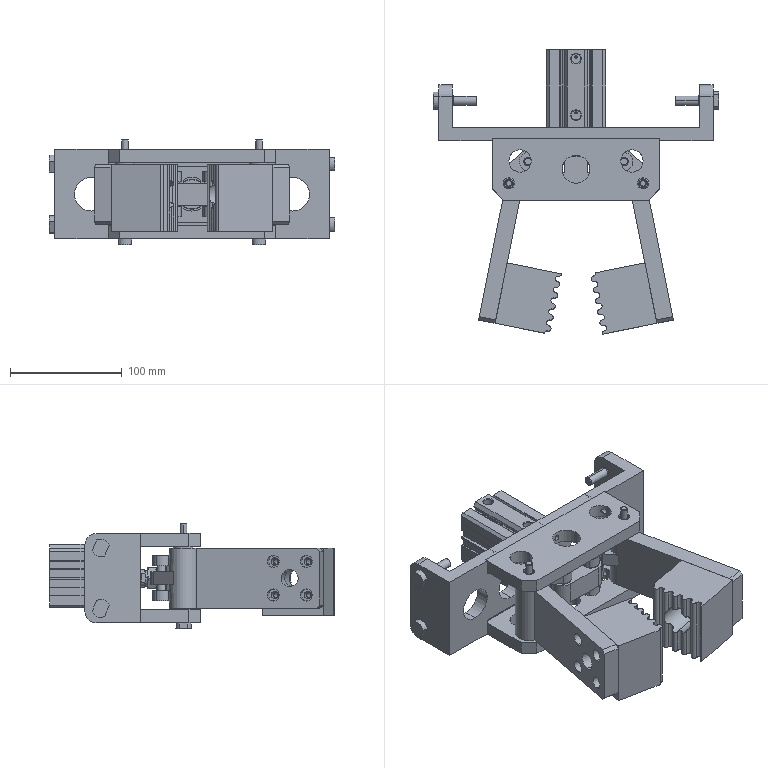Assembly | SolidWorks | mm | 29 component files | 29 solids | 997 faces | box 255 x 254.37 x 94 mm | volume 1114562 mm3 | cylinder 479 | plane 296 | cone 190 | torus 32 | commonest cylinder face diameters 5 x79 11 x40 10 x40 6.6 x36 8 x36 0.4 x35 16 x24 12 x24
Bill of materials:
ZTDJ-L-400-04-24-MaterialPortBagClamp-T-shapedConnectingRod | 1 | 1023 Carbon Steel Sheet (SS) | Prismatic block: an obround (stadium-shaped) body with two vertical through holes, one near each rounded end, plus a rectangular lug sticking out from one long side between the holes. The lug and the obround body look the same height.
C-SFF10120 | 4 | Tin Bronze | Flanged cylindrical sleeve: a thin circular flange on top of a straight cylindrical body, with one through bore along the axis.
MPBZ8_20 | 2 |  | Plain hollow cylindrical sleeve/tube with a straight through-bore and chamfered end edges; length roughly 1.6 times the outer diameter, and the bore is roughly two-thirds of the outer diameter (proportions estimated from the renders).
ZTDJ-01-20-AxisMountingPlate | 2 | 1023 Carbon Steel Sheet (SS) | Thin flat rectangular plate with two corners chamfered along one long edge. It has three large through holes in a row (the centre one is biggest) and two small through holes near the chamfered corners.
ZTDJ-L-400-04-16-MaterialPortBagClamp-Axis4 | 4 | 1023 Carbon Steel Sheet (SS) | Stepped cylindrical pin or shaft: a long smaller-diameter shank, a shorter larger-diameter section, and an end head that is wider still and has two parallel flats.
ZTDJ-L-400-04-19-MaterialPortBagClamp-ConnectingRodSeat2 | 1 | 1023 Carbon Steel Sheet (SS) | U-shaped channel bracket: a long rectangular web with a short perpendicular flange at each end. The web has five large through holes in a row and several small holes. Each flange has two holes and rounded outer corners.
ZTDJ-L-400-04-21-MaterialPortBagClamp-Axis5 | 2 | 1023 Carbon Steel Sheet (SS) | Slender stepped pin: a long main cylindrical body, a short smaller-diameter spigot at one end, and a wider collar or head at the other end with flats on its outline.
ZTDJ-L-400-04-22-MaterialPortBagClamp-BagClampingArm | 2 | 1023 Carbon Steel Sheet (SS) | Arm or lever-like bar: a long rectangular-section body with a round boss at one end carrying a through hole. A pattern of holes near the other end includes a larger central hole and four smaller holes, which appear counterbored.
ZTDJ-L-400-04-23-MaterialPortBagClamp-H-shapedConnectingRod | 2 | 1023 Carbon Steel Sheet (SS) | H-shaped part: two parallel obround plates, each with two through holes near the rounded ends, joined by a central rectangular web.
ZTDJ-L-400-04-25-MaterialPortBagClamp-Axis6 | 4 | Alloy Steel | Plain cylindrical pin with chamfered ends and two small radial holes, one near each end, on the same side.
ZTDJ-L-400-04-26-MaterialPortBagClamp-BagClampingAluminumBlock | 2 | 6061-T6 (SS) | Rectangular block with a row of semicircular scallops along one edge (they run as grooves along its full length). One face has a large round through bore with four small holes in a square pattern around it.
Mates:
1. coincident | ZTDJ-L-400-04-19-MaterialPortBagClamp-ConnectingRodSeat2-1 face at (-28.439, -44.186, 290) dir (0, -1, 0) | ZTDJ-01-20-AxisMountingPlate-1 face at (-103.439, -44.186, 330) dir (0, 1, 0)
2. coincident | ZTDJ-L-400-04-19-MaterialPortBagClamp-ConnectingRodSeat2-1 plane at (-28.439, -46.186, 290) dir (1, 0, 0) | ZTDJ-01-20-AxisMountingPlate-1 plane at (-28.439, -71.686, 324) dir (1, 0, 0)
3. coincident | ZTDJ-L-400-04-19-MaterialPortBagClamp-ConnectingRodSeat2-1 face at (-28.439, -44.186, 290) dir (0, -1, 0) | ZTDJ-01-20-AxisMountingPlate-2 face at (-103.439, -44.186, 262) dir (0, 1, 0)
4. coincident | ZTDJ-L-400-04-19-MaterialPortBagClamp-ConnectingRodSeat2-1 plane at (-28.439, -46.186, 290) dir (1, 0, 0) | ZTDJ-01-20-AxisMountingPlate-2 plane at (-28.439, -71.686, 256) dir (1, 0, 0)
5. concentric | ZTDJ-01-20-AxisMountingPlate-1 face at (31.561, -84.186, 318) dir (0, 0, 1) r 5 | ZTDJ-L-400-04-22-MaterialPortBagClamp-BagClampingArm-1 face at (31.561, -84.186, 263) dir (0, 0, 1) r 5.5
6. concentric | ZTDJ-01-20-AxisMountingPlate-2 face at (-88.439, -84.186, 250) dir (0, 0, 1) r 5 | ZTDJ-L-400-04-22-MaterialPortBagClamp-BagClampingArm-2 face at (-88.439, -84.186, 317) dir (0, 0, -1) r 5.5
7. concentric | ZTDJ-L-400-04-23-MaterialPortBagClamp-H-shapedConnectingRod-2 face at (-71.256, -64.673, 310) dir (0, 0, -1) r 4 | ZTDJ-L-400-04-22-MaterialPortBagClamp-BagClampingArm-2 face at (-71.256, -64.673, 296) dir (0, 0, -1) r 5
8. concentric | ZTDJ-L-400-04-19-MaterialPortBagClamp-ConnectingRodSeat2-1 face at (-28.439, 3.814, 290) dir (0, -1, 0) r 15 | ACQ40x30SB(0)+()-1/ACQS-40x30-B_30r-1 face at (-28.439, 18.755, 290) dir (0, -1, 0) r 8
9. coincident | ZTDJ-L-400-04-19-MaterialPortBagClamp-ConnectingRodSeat2-1 face at (-28.439, -34.186, 290) dir (0, 1, 0) | ACQ40x30SB(0)+()-1/ACQS-40x3030_b-1 face at (-20.039, -34.186, 264.2) dir (0, -1, 0)
10. coincident | ZTDJ-L-400-04-19-MaterialPortBagClamp-ConnectingRodSeat2-1 face at (-150.939, -34.186, 250) dir (0, 0, -1) | ZTDJ-01-20-AxisMountingPlate-2 face at (-28.439, -71.686, 250) dir (0, 0, -1)
11. coincident | ZTDJ-L-400-04-19-MaterialPortBagClamp-ConnectingRodSeat2-1 face at (34.061, -34.186, 330) dir (0, 0, 1) | ZTDJ-01-20-AxisMountingPlate-1 face at (-28.439, -71.686, 330) dir (0, 0, 1)
12. concentric | ZTDJ-L-400-04-23-MaterialPortBagClamp-H-shapedConnectingRod-2 face at (-45.939, -84.245, 310) dir (0, 0, -1) r 4 | ACQ40x30SB(0)+()-1/ZTDJ-L-400-04-24-MaterialPortBagClamp-T-shapedConnectingRod-2 face at (-45.939, -84.245, 300) dir (0, 0, -1) r 6
13. concentric | ZTDJ-L-400-04-23-MaterialPortBagClamp-H-shapedConnectingRod-1 face at (-10.939, -84.245, 310) dir (0, 0, -1) r 4 | ACQ40x30SB(0)+()-1/ZTDJ-L-400-04-24-MaterialPortBagClamp-T-shapedConnectingRod-2 face at (-10.939, -84.245, 300) dir (0, 0, -1) r 6
14. concentric | ZTDJ-L-400-04-22-MaterialPortBagClamp-BagClampingArm-1 face at (14.378, -64.673, 284) dir (0, 0, 1) r 5 | ZTDJ-L-400-04-23-MaterialPortBagClamp-H-shapedConnectingRod-1 face at (14.378, -64.673, 310) dir (0, 0, -1) r 4
15. distance | ZTDJ-L-400-04-23-MaterialPortBagClamp-H-shapedConnectingRod-2 face at (-82.478, -66.11, 279) dir (0, 0, 1) | ACQ40x30SB(0)+()-1/ZTDJ-L-400-04-24-MaterialPortBagClamp-T-shapedConnectingRod-2 face at (-45.939, -84.245, 280) dir (0, 0, -1)
16. coincident | ZTDJ-L-400-04-23-MaterialPortBagClamp-H-shapedConnectingRod-1 face at (-10.939, -84.245, 270) dir (0, 0, -1) | ZTDJ-L-400-04-23-MaterialPortBagClamp-H-shapedConnectingRod-2 face at (-71.256, -64.673, 270) dir (0, 0, -1)
17. concentric | ZTDJ-L-400-04-19-MaterialPortBagClamp-ConnectingRodSeat2-1 face at (-150.939, -10.186, 263) dir (1, 0, 0) r 5 | ZTDJ-L-400-04-16-MaterialPortBagClamp-Axis4-4 face at (-150.939, -10.186, 263) dir (1, 0, 0) r 5
18. coincident | ZTDJ-L-400-04-19-MaterialPortBagClamp-ConnectingRodSeat2-1 face at (-150.939, -34.186, 330) dir (-1, 0, 0) | ZTDJ-L-400-04-16-MaterialPortBagClamp-Axis4-4 face at (-150.939, -10.186, 263) dir (1, 0, 0)
19. concentric | ZTDJ-L-400-04-19-MaterialPortBagClamp-ConnectingRodSeat2-1 face at (-150.939, -10.186, 317) dir (1, 0, 0) r 5 | ZTDJ-L-400-04-16-MaterialPortBagClamp-Axis4-3 face at (-150.939, -10.186, 317) dir (1, 0, 0) r 5
20. coincident | ZTDJ-L-400-04-16-MaterialPortBagClamp-Axis4-3 face at (-155.939, -10.186, 317) dir (-1, 0, 0) | ZTDJ-L-400-04-16-MaterialPortBagClamp-Axis4-4 face at (-155.939, -10.186, 263) dir (-1, 0, 0)
21. concentric | ZTDJ-L-400-04-19-MaterialPortBagClamp-ConnectingRodSeat2-1 face at (-150.939, -10.186, 263) dir (1, 0, 0) r 5 | ZTDJ-L-400-04-16-MaterialPortBagClamp-Axis4-2 face at (94.061, -10.186, 263) dir (-1, 0, 0) r 5
22. concentric | ZTDJ-L-400-04-19-MaterialPortBagClamp-ConnectingRodSeat2-1 face at (-150.939, -10.186, 317) dir (1, 0, 0) r 5 | ZTDJ-L-400-04-16-MaterialPortBagClamp-Axis4-1 face at (94.061, -10.186, 317) dir (-1, 0, 0) r 5
23. coincident | ZTDJ-L-400-04-19-MaterialPortBagClamp-ConnectingRodSeat2-1 face at (94.061, -34.186, 330) dir (1, 0, 0) | ZTDJ-L-400-04-16-MaterialPortBagClamp-Axis4-2 face at (94.061, -10.186, 263) dir (-1, 0, 0)
24. coincident | ZTDJ-L-400-04-19-MaterialPortBagClamp-ConnectingRodSeat2-1 face at (94.061, -34.186, 330) dir (1, 0, 0) | ZTDJ-L-400-04-16-MaterialPortBagClamp-Axis4-1 face at (94.061, -10.186, 317) dir (-1, 0, 0)
25. concentric | ACQ40x30SB(0)+()-1/ZTDJ-L-400-04-24-MaterialPortBagClamp-T-shapedConnectingRod-2 face at (-10.939, -84.245, 300) dir (0, 0, -1) r 6 | MPBZ8_20-1 face at (-10.939, -84.245, 280) dir (0, 0, 1) r 6
26. coincident | ACQ40x30SB(0)+()-1/ZTDJ-L-400-04-24-MaterialPortBagClamp-T-shapedConnectingRod-2 face at (-45.939, -84.245, 300) dir (0, 0, 1) | MPBZ8_20-1 face at (-15.171, -88.063, 300) dir (0, 0, 1)
27. concentric | ACQ40x30SB(0)+()-1/ZTDJ-L-400-04-24-MaterialPortBagClamp-T-shapedConnectingRod-2 face at (-45.939, -84.245, 300) dir (0, 0, -1) r 6 | MPBZ8_20-2 face at (-45.939, -84.245, 280) dir (0, 0, 1) r 6
28. coincident | ACQ40x30SB(0)+()-1/ZTDJ-L-400-04-24-MaterialPortBagClamp-T-shapedConnectingRod-2 face at (-45.939, -84.245, 300) dir (0, 0, 1) | MPBZ8_20-2 face at (-46.858, -78.62, 300) dir (0, 0, 1)
29. concentric | ZTDJ-L-400-04-23-MaterialPortBagClamp-H-shapedConnectingRod-1 face at (14.378, -64.673, 310) dir (0, 0, -1) r 4 | ZTDJ-L-400-04-25-MaterialPortBagClamp-Axis6-1 face at (14.378, -64.673, 310) dir (0, 0, -1) r 4
30. concentric | ZTDJ-L-400-04-23-MaterialPortBagClamp-H-shapedConnectingRod-1 face at (-10.939, -84.245, 310) dir (0, 0, -1) r 4 | ZTDJ-L-400-04-25-MaterialPortBagClamp-Axis6-2 face at (-10.939, -84.245, 310) dir (0, 0, -1) r 4
31. concentric | ZTDJ-L-400-04-23-MaterialPortBagClamp-H-shapedConnectingRod-2 face at (-45.939, -84.245, 310) dir (0, 0, -1) r 4 | ZTDJ-L-400-04-25-MaterialPortBagClamp-Axis6-3 face at (-45.939, -84.245, 310) dir (0, 0, -1) r 4
32. concentric | ZTDJ-L-400-04-23-MaterialPortBagClamp-H-shapedConnectingRod-2 face at (-71.256, -64.673, 310) dir (0, 0, -1) r 4 | ZTDJ-L-400-04-25-MaterialPortBagClamp-Axis6-4 face at (-71.256, -64.673, 310) dir (0, 0, -1) r 4
33. concentric | ZTDJ-01-20-AxisMountingPlate-2 face at (31.561, -84.186, 250) dir (0, 0, 1) r 5 | ZTDJ-L-400-04-21-MaterialPortBagClamp-Axis5-1 face at (31.561, -84.186, 329) dir (0, 0, -1) r 5
34. coincident | ZTDJ-01-20-AxisMountingPlate-2 face at (-28.439, -71.686, 250) dir (0, 0, -1) | ZTDJ-L-400-04-21-MaterialPortBagClamp-Axis5-1 face at (31.561, -84.186, 250) dir (0, 0, 1)
35. concentric | ZTDJ-01-20-AxisMountingPlate-1 face at (-88.439, -84.186, 318) dir (0, 0, 1) r 5 | ZTDJ-L-400-04-21-MaterialPortBagClamp-Axis5-2 face at (-88.439, -84.186, 329) dir (0, 0, -1) r 5
36. coincident | ZTDJ-01-20-AxisMountingPlate-2 face at (-28.439, -71.686, 250) dir (0, 0, -1) | ZTDJ-L-400-04-21-MaterialPortBagClamp-Axis5-2 face at (-88.439, -84.186, 250) dir (0, 0, 1)
37. coincident | ZTDJ-L-400-04-22-MaterialPortBagClamp-BagClampingArm-1 face at (22.263, -101.355, 137.103) dir (-0.9804, -0.1971, 0) | ZTDJ-L-400-04-26-MaterialPortBagClamp-BagClampingAluminumBlock-1 face at (33.103, -155.277, 257) dir (0.9804, 0.1971, 0)
38. coincident | ZTDJ-L-400-04-22-MaterialPortBagClamp-BagClampingArm-2 face at (-79.141, -101.355, 442.897) dir (0.9804, -0.1971, 0) | ZTDJ-L-400-04-26-MaterialPortBagClamp-BagClampingAluminumBlock-2 face at (-100.821, -209.198, 257) dir (-0.9804, 0.1971, 0)
39. coincident | ZTDJ-L-400-04-22-MaterialPortBagClamp-BagClampingArm-2 face at (-88.439, -84.186, 317) dir (0, 0, 1) | ZTDJ-L-400-04-26-MaterialPortBagClamp-BagClampingAluminumBlock-2 face at (-72.117, -186.918, 317) dir (0, 0, 1)
40. distance | ZTDJ-L-400-04-22-MaterialPortBagClamp-BagClampingArm-2 face at (-100.821, -209.198, 442.897) dir (-0.1971, -0.9804, 0) | ZTDJ-L-400-04-26-MaterialPortBagClamp-BagClampingAluminumBlock-2 face at (-54.253, -218.56, 257) dir (-0.1971, -0.9804, 0)
41. concentric | ZTDJ-L-400-04-22-MaterialPortBagClamp-BagClampingArm-1 face at (31.561, -84.186, 302) dir (0, 0, 1) r 6 | C-SFF10120-1 face at (31.561, -84.186, 318) dir (0, 0, 1) r 6
42. coincident | ZTDJ-L-400-04-22-MaterialPortBagClamp-BagClampingArm-1 face at (31.561, -84.186, 317) dir (0, 0, 1) | C-SFF10120-1 face at (31.561, -75.186, 317) dir (0, 0, -1)
43. concentric | ZTDJ-L-400-04-22-MaterialPortBagClamp-BagClampingArm-1 face at (31.561, -84.186, 278) dir (0, 0, -1) r 6 | C-SFF10120-2 face at (31.561, -84.186, 262) dir (0, 0, -1) r 6
44. coincident | ZTDJ-L-400-04-22-MaterialPortBagClamp-BagClampingArm-1 face at (31.561, -84.186, 263) dir (0, 0, -1) | C-SFF10120-2 face at (28.114, -75.872, 263) dir (0, 0, 1)
45. coincident | ZTDJ-L-400-04-22-MaterialPortBagClamp-BagClampingArm-2 face at (-88.439, -84.186, 263) dir (0, 0, -1) | C-SFF10120-3 face at (-91.886, -75.872, 263) dir (0, 0, 1)
46. concentric | ZTDJ-L-400-04-22-MaterialPortBagClamp-BagClampingArm-2 face at (-88.439, -84.186, 278) dir (0, 0, -1) r 6 | C-SFF10120-3 face at (-88.439, -84.186, 262) dir (0, 0, -1) r 6
47. coincident | ZTDJ-L-400-04-22-MaterialPortBagClamp-BagClampingArm-2 face at (-88.439, -84.186, 317) dir (0, 0, 1) | C-SFF10120-4 face at (-88.439, -75.186, 317) dir (0, 0, -1)
48. concentric | ZTDJ-L-400-04-22-MaterialPortBagClamp-BagClampingArm-2 face at (-88.439, -84.186, 302) dir (0, 0, 1) r 6 | C-SFF10120-4 face at (-88.439, -84.186, 318) dir (0, 0, 1) r 6
49. coincident | ZTDJ-01-20-AxisMountingPlate-2 face at (-28.439, -71.686, 262) dir (0, 0, 1) | C-SFF10120-3 face at (-90.354, -79.567, 262) dir (0, 0, -1)
50. coincident | ZTDJ-01-20-AxisMountingPlate-1 face at (-28.439, -71.686, 318) dir (0, 0, -1) | C-SFF10120-1 face at (31.561, -79.186, 318) dir (0, 0, 1)
51. coincident | ZTDJ-L-400-04-22-MaterialPortBagClamp-BagClampingArm-1 face at (43.944, -209.198, 137.103) dir (0.1971, -0.9804, 0) | ZTDJ-L-400-04-26-MaterialPortBagClamp-BagClampingAluminumBlock-1 face at (-2.625, -218.56, 257) dir (0.1971, -0.9804, 0)
52. coincident | ZTDJ-L-400-04-22-MaterialPortBagClamp-BagClampingArm-1 face at (31.561, -84.186, 317) dir (0, 0, 1) | ZTDJ-L-400-04-26-MaterialPortBagClamp-BagClampingAluminumBlock-1 face at (15.239, -186.918, 317) dir (0, 0, 1)
53. coincident | ZTDJ-L-400-04-23-MaterialPortBagClamp-H-shapedConnectingRod-1 face at (-10.939, -84.245, 270) dir (0, 0, -1) | ZTDJ-L-400-04-25-MaterialPortBagClamp-Axis6-1 face at (14.378, -64.673, 270) dir (0, 0, -1)
54. coincident | ZTDJ-L-400-04-23-MaterialPortBagClamp-H-shapedConnectingRod-2 face at (-71.256, -64.673, 270) dir (0, 0, -1) | ZTDJ-L-400-04-25-MaterialPortBagClamp-Axis6-4 face at (-71.256, -64.673, 270) dir (0, 0, -1)
55. coincident | ZTDJ-L-400-04-23-MaterialPortBagClamp-H-shapedConnectingRod-2 face at (-71.256, -64.673, 270) dir (0, 0, -1) | ZTDJ-L-400-04-25-MaterialPortBagClamp-Axis6-3 face at (-45.939, -84.245, 270) dir (0, 0, -1)
56. coincident | ZTDJ-L-400-04-23-MaterialPortBagClamp-H-shapedConnectingRod-1 face at (-10.939, -84.245, 270) dir (0, 0, -1) | ZTDJ-L-400-04-25-MaterialPortBagClamp-Axis6-2 face at (-10.939, -84.245, 270) dir (0, 0, -1)
57. distance | ACQS-40x30-B_30r-1 face at (-58.5, 0, 0) dir (-1, 0, 0) | ACQS-40x3030_b-1 face at (0, -8.4, -25.8) dir (-1, 0, 0)
58. concentric | ACQS-40x3030_b-1 face at (64.5, 0, 0) dir (-1, 0, 0) r 8 | ACQS-40x30-B_30r-1 face at (34.5, 0, 0) dir (-1, 0, 0) r 8
59. concentric | ACQS-40x30-B_30r-1 face at (-30, 0, 0) dir (-1, 0, 0) r 7 | ACQ 40_Nut-1 face at (-44.5, 0, 0) dir (1, 0, 0) r 6.188
60. distance | ACQ 40_Nut-1 face at (-44.5, -9.5, 0) dir (-1, 0, 0) | ACQS-40x30-B_30r-1 face at (-58.5, 0, 0) dir (-1, 0, 0)
61. concentric | ACQS-40x30-B_30r-1 face at (-30, 0, 0) dir (-1, 0, 0) r 7 | ZTDJ-L-400-04-24-MaterialPortBagClamp-T-shapedConnectingRod-2 face at (-44.5, 0, 0) dir (1, 0, 0) r 7
62. coincident | ACQ 40_Nut-1 face at (-44.5, -9.5, 0) dir (-1, 0, 0) | ZTDJ-L-400-04-24-MaterialPortBagClamp-T-shapedConnectingRod-2 face at (-44.5, 0, 0) dir (1, 0, 0)